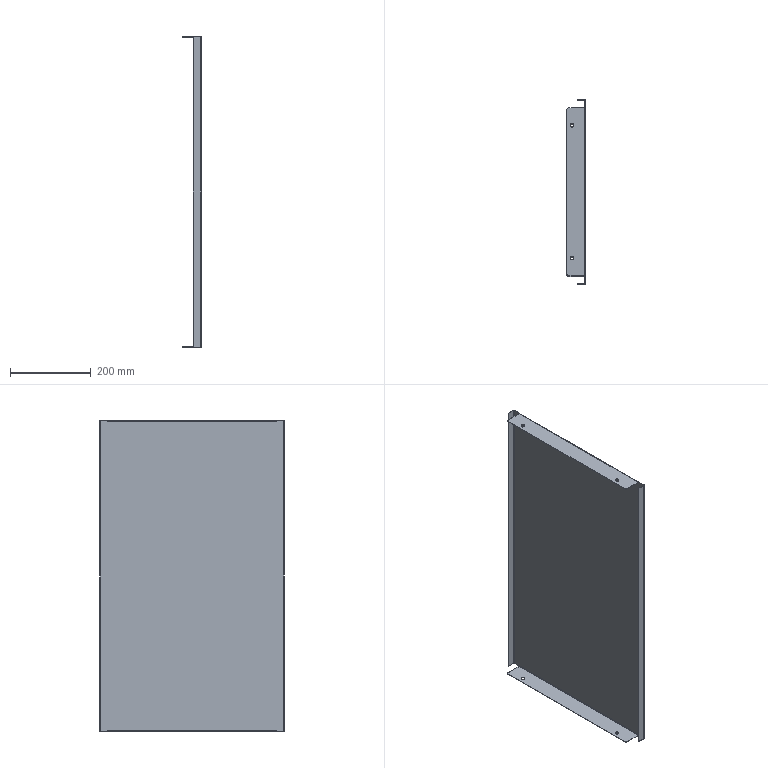Component | SolidWorks | UpperLeftSidePlate-1_UpperLeftOuterSidePanel-1 | 1 solid | 66 faces | volume 334609 mm3 | plane 46 | cylinder 20 | commonest cylinder face diameters 9 x8 3.6 x4 2 x4 10 x4 | material 304